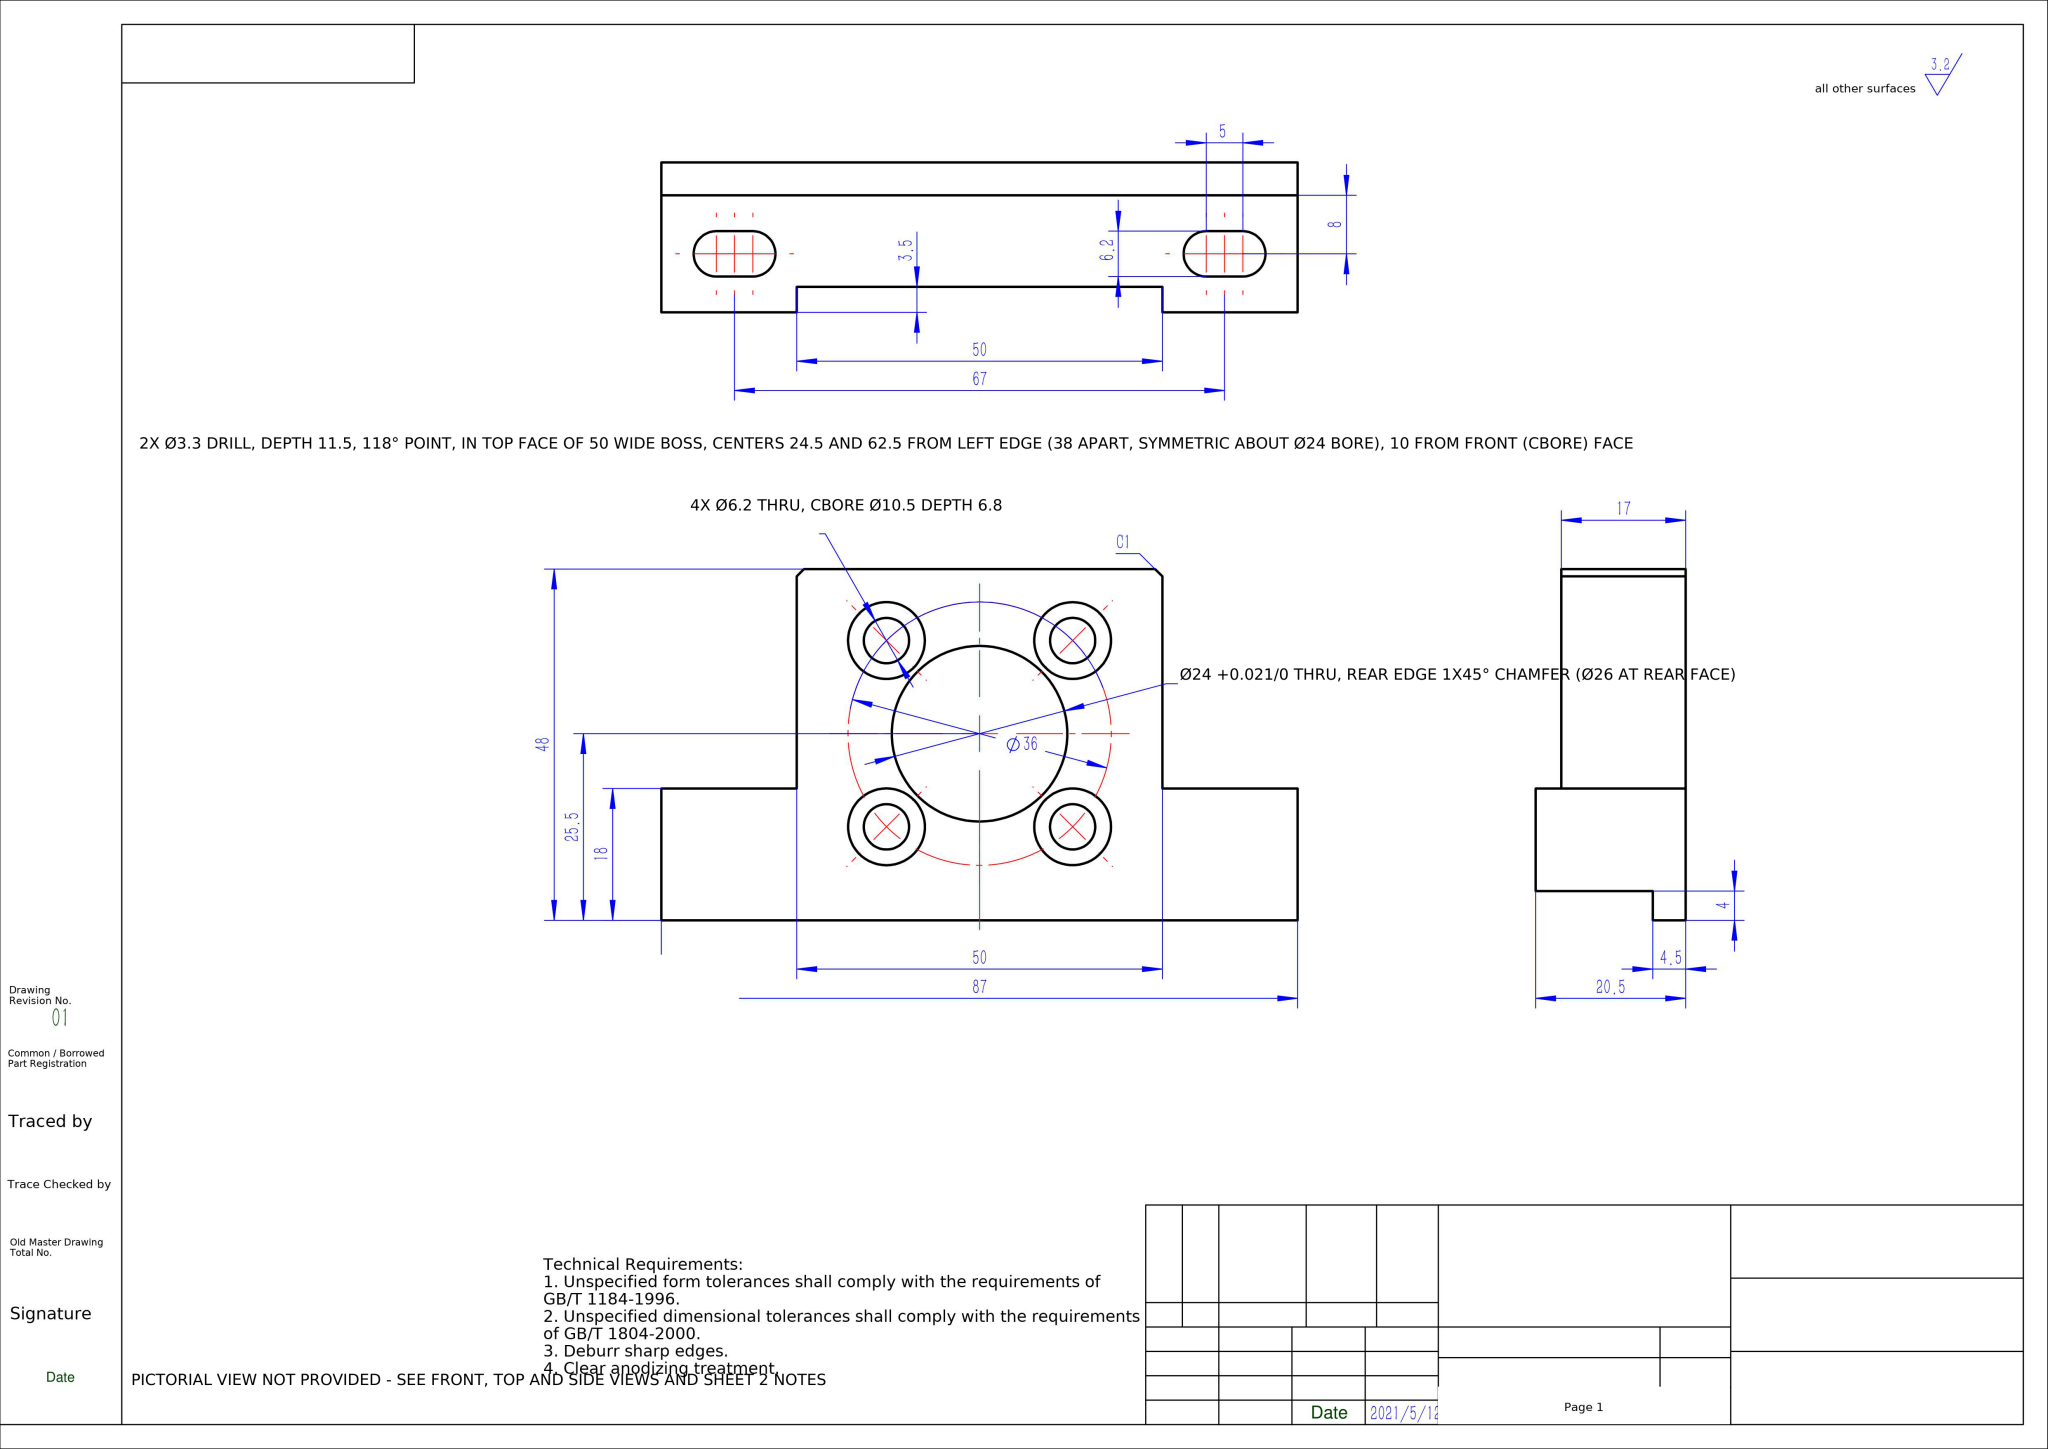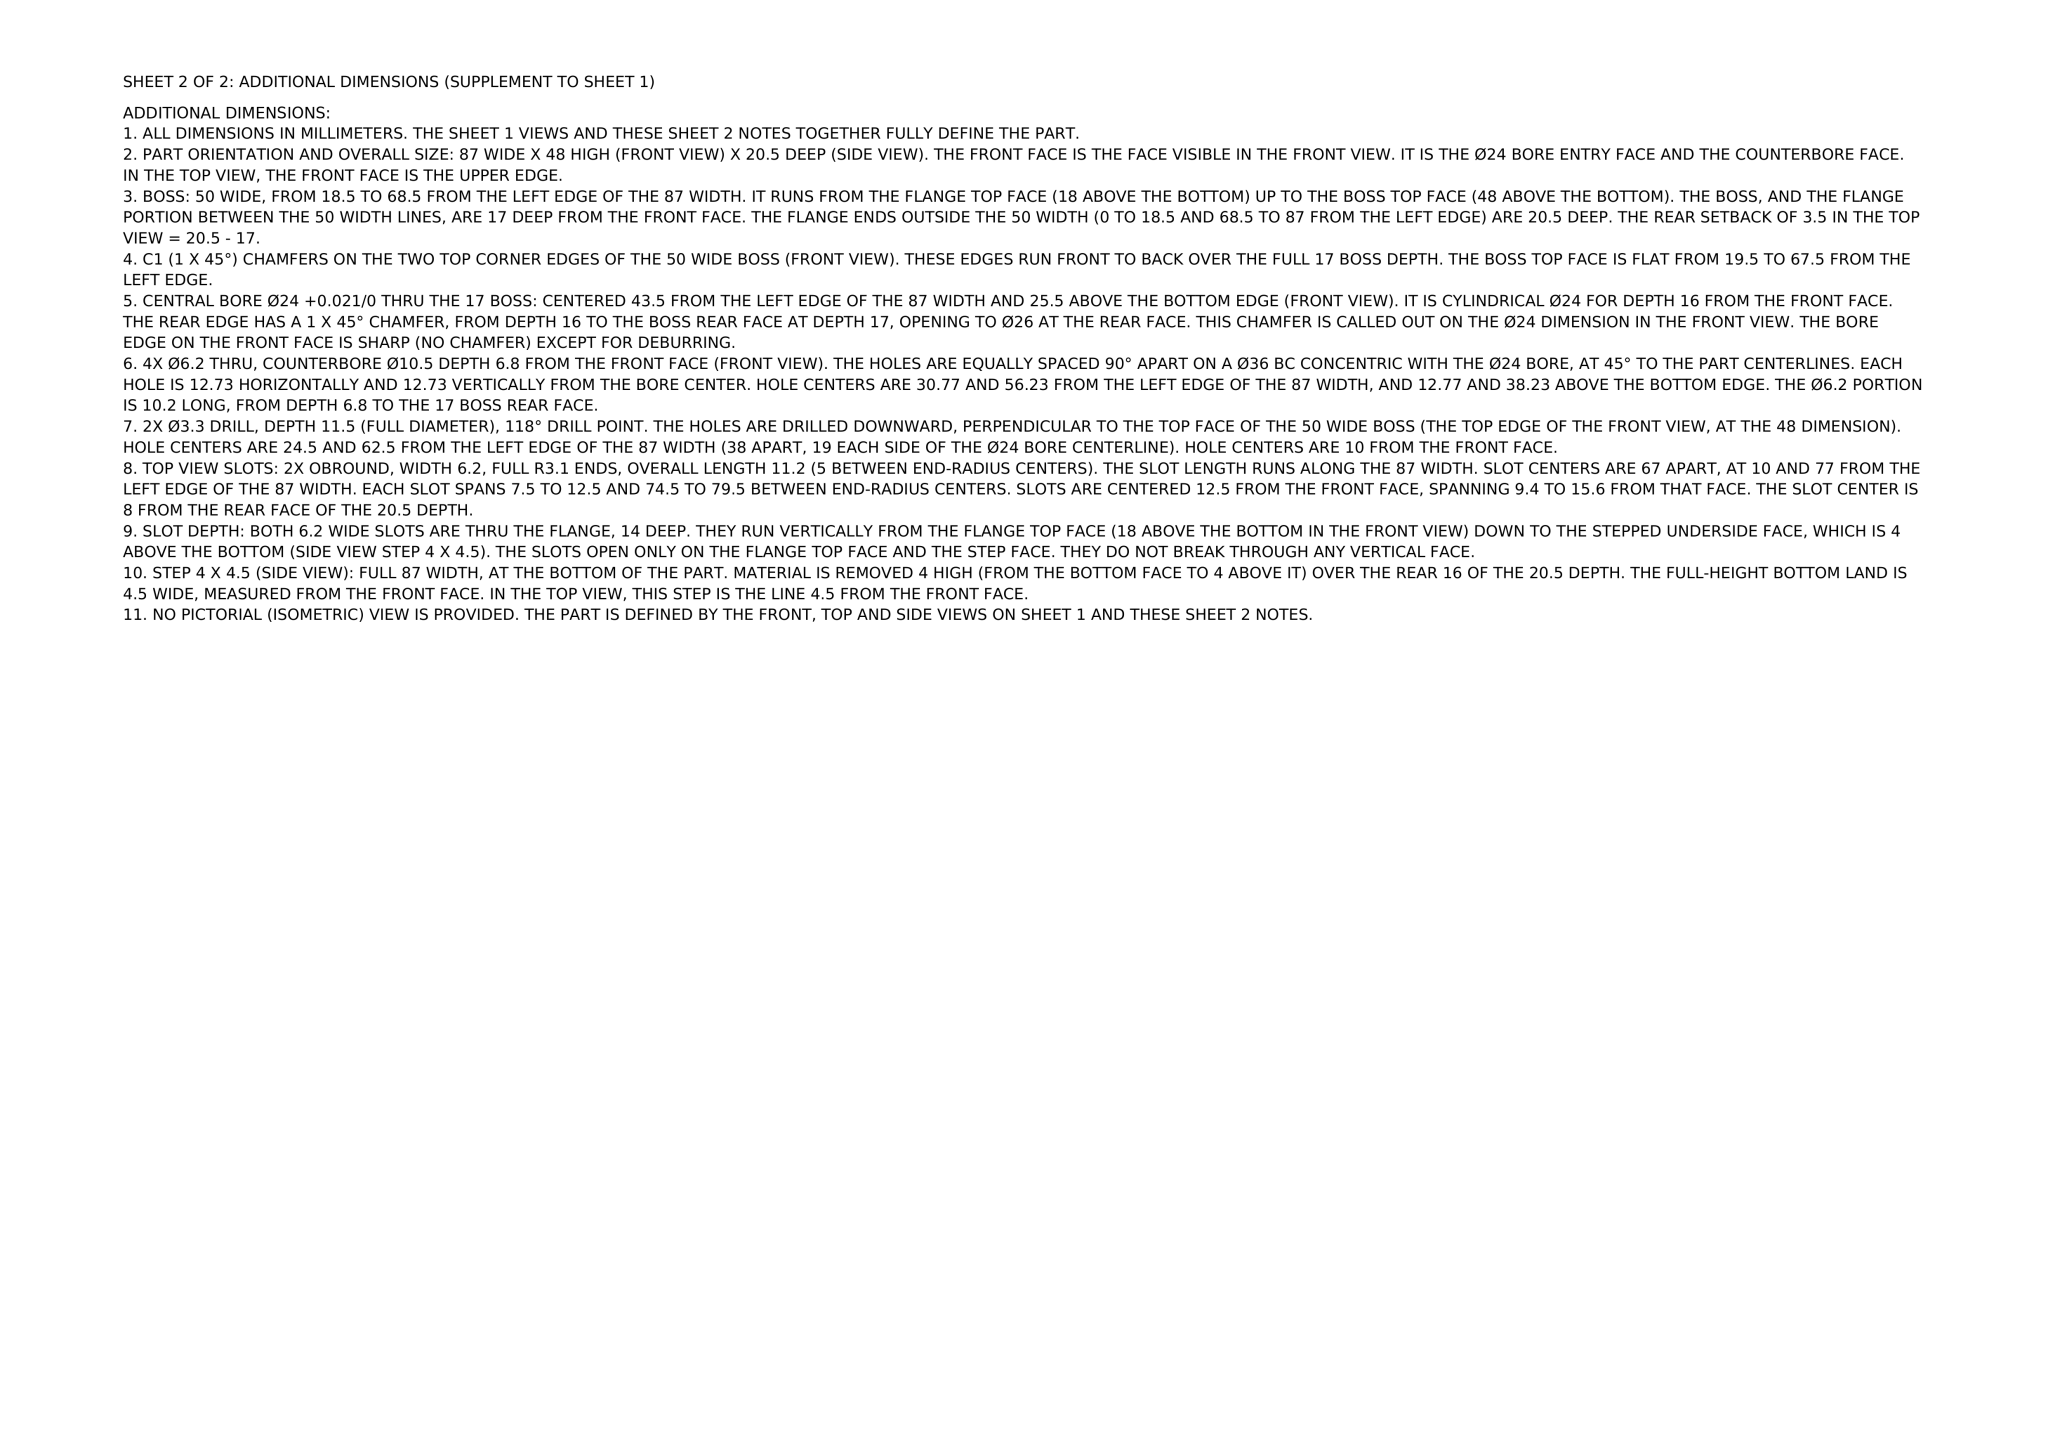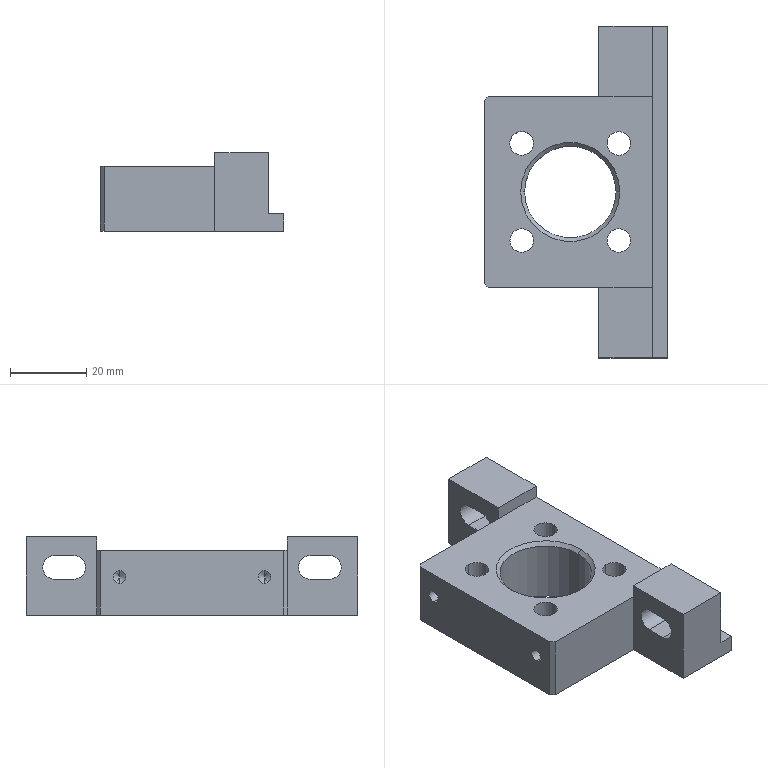Part | NX | mm | 1 solid | 58 faces | box 48 x 87 x 20.5 mm | volume 36336 mm3 | cylinder 26 | plane 26 | cone 6 | commonest cylinder face diameters 6.2 x12 10.5 x8 3.3 x4 24 x2